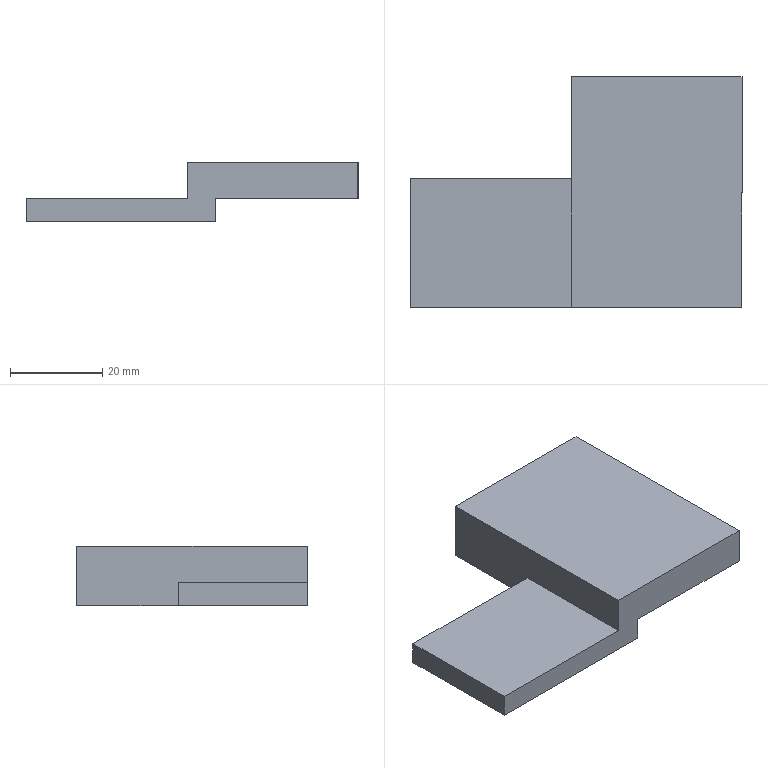Component | SolidWorks | MirroredGripper-2024-3-4-06-2 | 1 solid | 11 faces | box 72 x 50 x 13 mm | volume 21200 mm3 | plane 11 | material S45C
STEP:
#1=COLOUR_RGB('',0.7922,0.8196,0.9333);
#2=FILL_AREA_STYLE_COLOUR('',#1);
#3=FILL_AREA_STYLE('',(#2));
#4=SURFACE_STYLE_FILL_AREA(#3);
#5=SURFACE_SIDE_STYLE('',(#4));
#6=SURFACE_STYLE_USAGE(.BOTH.,#5);
#7=PRESENTATION_STYLE_ASSIGNMENT((#6));
#8=CARTESIAN_POINT('',(-6.049,-0.2645,10.276));
#9=VERTEX_POINT('',#8);
#10=CARTESIAN_POINT('',(-6.049,0.8378,10.276));
#11=VERTEX_POINT('',#10);
#12=CARTESIAN_POINT('',(-6.049,-0.2645,10.276));
#13=DIRECTION('',(0.,1.,-0.));
#14=VECTOR('',#13,39.37);
#15=LINE('',#12,#14);
#16=EDGE_CURVE('',#9,#11,#15,.T.);
#17=ORIENTED_EDGE('',*,*,#16,.F.);
#18=CARTESIAN_POINT('',(-6.049,-0.2645,10.472));
#19=VERTEX_POINT('',#18);
#20=CARTESIAN_POINT('',(-6.049,-0.2645,10.472));
#21=DIRECTION('',(-0.,0.,1.));
#22=VECTOR('',#21,39.37);
#23=LINE('',#20,#22);
#24=EDGE_CURVE('',#9,#19,#23,.T.);
#25=ORIENTED_EDGE('',*,*,#24,.T.);
#26=CARTESIAN_POINT('',(-6.049,0.8378,10.472));
#27=VERTEX_POINT('',#26);
#28=CARTESIAN_POINT('',(-6.049,-0.2645,10.472));
#29=DIRECTION('',(0.,1.,-0.));
#30=VECTOR('',#29,39.37);
#31=LINE('',#28,#30);
#32=EDGE_CURVE('',#19,#27,#31,.T.);
#33=ORIENTED_EDGE('',*,*,#32,.T.);
#34=CARTESIAN_POINT('',(-6.049,0.8378,11.85));
#35=DIRECTION('',(0.,-0.,-1.));
#36=VECTOR('',#35,39.37);
#37=LINE('',#34,#36);
#38=EDGE_CURVE('',#27,#11,#37,.T.);
#39=ORIENTED_EDGE('',*,*,#38,.T.);
#40=EDGE_LOOP('',(#17,#25,#33,#39));
#41=FACE_OUTER_BOUND('',#40,.T.);
#42=CARTESIAN_POINT('',(-6.049,-0.2645,10.472));
#43=DIRECTION('',(1.,-0.,0.));
#44=DIRECTION('',(0.,1.,-0.));
#45=AXIS2_PLACEMENT_3D('',#42,#43,#44);
#46=PLANE('',#45);
#47=ADVANCED_FACE('',(#41),#46,.F.);
#48=ORIENTED_EDGE('',*,*,#32,.F.);
#49=CARTESIAN_POINT('',(-4.671,-0.2645,10.472));
#50=VERTEX_POINT('',#49);
#51=CARTESIAN_POINT('',(-6.049,-0.2645,10.472));
#52=DIRECTION('',(1.,-0.,0.));
#53=VECTOR('',#52,39.37);
#54=LINE('',#51,#53);
#55=EDGE_CURVE('',#19,#50,#54,.T.);
#56=ORIENTED_EDGE('',*,*,#55,.T.);
#57=CARTESIAN_POINT('',(-4.671,0.8378,10.472));
#58=VERTEX_POINT('',#57);
#59=CARTESIAN_POINT('',(-4.671,-0.2645,10.472));
#60=DIRECTION('',(0.,1.,-0.));
#61=VECTOR('',#60,39.37);
#62=LINE('',#59,#61);
#63=EDGE_CURVE('',#50,#58,#62,.T.);
#64=ORIENTED_EDGE('',*,*,#63,.T.);
#65=CARTESIAN_POINT('',(-6.049,0.8378,10.472));
#66=DIRECTION('',(1.,-0.,0.));
#67=VECTOR('',#66,39.37);
#68=LINE('',#65,#67);
#69=EDGE_CURVE('',#27,#58,#68,.T.);
#70=ORIENTED_EDGE('',*,*,#69,.F.);
#71=EDGE_LOOP('',(#48,#56,#64,#70));
#72=FACE_OUTER_BOUND('',#71,.T.);
#73=CARTESIAN_POINT('',(-6.049,-0.2645,10.472));
#74=DIRECTION('',(0.,-0.,-1.));
#75=DIRECTION('',(-0.,-1.,0.));
#76=AXIS2_PLACEMENT_3D('',#73,#74,#75);
#77=PLANE('',#76);
#78=ADVANCED_FACE('',(#72),#77,.F.);
#79=ORIENTED_EDGE('',*,*,#63,.F.);
#80=CARTESIAN_POINT('',(-4.671,-0.2645,10.787));
#81=VERTEX_POINT('',#80);
#82=CARTESIAN_POINT('',(-4.671,-0.2645,10.472));
#83=DIRECTION('',(-0.,0.,1.));
#84=VECTOR('',#83,39.37);
#85=LINE('',#82,#84);
#86=EDGE_CURVE('',#50,#81,#85,.T.);
#87=ORIENTED_EDGE('',*,*,#86,.T.);
#88=CARTESIAN_POINT('',(-4.671,1.704,10.787));
#89=VERTEX_POINT('',#88);
#90=CARTESIAN_POINT('',(-4.671,-0.2645,10.787));
#91=DIRECTION('',(0.,1.,-0.));
#92=VECTOR('',#91,39.37);
#93=LINE('',#90,#92);
#94=EDGE_CURVE('',#81,#89,#93,.T.);
#95=ORIENTED_EDGE('',*,*,#94,.T.);
#96=CARTESIAN_POINT('',(-4.671,1.704,10.276));
#97=VERTEX_POINT('',#96);
#98=CARTESIAN_POINT('',(-4.671,1.704,10.472));
#99=DIRECTION('',(-0.,0.,1.));
#100=VECTOR('',#99,39.37);
#101=LINE('',#98,#100);
#102=EDGE_CURVE('',#97,#89,#101,.T.);
#103=ORIENTED_EDGE('',*,*,#102,.F.);
#104=CARTESIAN_POINT('',(-4.671,0.8378,10.276));
#105=VERTEX_POINT('',#104);
#106=CARTESIAN_POINT('',(-4.671,1.704,10.276));
#107=DIRECTION('',(0.,1.,-0.));
#108=VECTOR('',#107,39.37);
#109=LINE('',#106,#108);
#110=EDGE_CURVE('',#105,#97,#109,.T.);
#111=ORIENTED_EDGE('',*,*,#110,.F.);
#112=CARTESIAN_POINT('',(-4.671,0.8378,11.85));
#113=DIRECTION('',(0.,-0.,-1.));
#114=VECTOR('',#113,39.37);
#115=LINE('',#112,#114);
#116=EDGE_CURVE('',#58,#105,#115,.T.);
#117=ORIENTED_EDGE('',*,*,#116,.F.);
#118=EDGE_LOOP('',(#79,#87,#95,#103,#111,#117));
#119=FACE_OUTER_BOUND('',#118,.T.);
#120=CARTESIAN_POINT('',(-4.671,-0.2645,10.472));
#121=DIRECTION('',(1.,-0.,0.));
#122=DIRECTION('',(0.,1.,-0.));
#123=AXIS2_PLACEMENT_3D('',#120,#121,#122);
#124=PLANE('',#123);
#125=ADVANCED_FACE('',(#119),#124,.F.);
#126=CARTESIAN_POINT('',(-3.215,1.704,10.787));
#127=VERTEX_POINT('',#126);
#128=CARTESIAN_POINT('',(-4.671,1.704,10.787));
#129=DIRECTION('',(1.,-0.,0.));
#130=VECTOR('',#129,39.37);
#131=LINE('',#128,#130);
#132=EDGE_CURVE('',#89,#127,#131,.T.);
#133=ORIENTED_EDGE('',*,*,#132,.F.);
#134=ORIENTED_EDGE('',*,*,#94,.F.);
#135=CARTESIAN_POINT('',(-3.215,-0.2645,10.787));
#136=VERTEX_POINT('',#135);
#137=CARTESIAN_POINT('',(-4.671,-0.2645,10.787));
#138=DIRECTION('',(1.,-0.,0.));
#139=VECTOR('',#138,39.37);
#140=LINE('',#137,#139);
#141=EDGE_CURVE('',#81,#136,#140,.T.);
#142=ORIENTED_EDGE('',*,*,#141,.T.);
#143=CARTESIAN_POINT('',(-3.215,-0.2645,10.787));
#144=DIRECTION('',(0.,1.,-0.));
#145=VECTOR('',#144,39.37);
#146=LINE('',#143,#145);
#147=EDGE_CURVE('',#136,#127,#146,.T.);
#148=ORIENTED_EDGE('',*,*,#147,.T.);
#149=EDGE_LOOP('',(#133,#134,#142,#148));
#150=FACE_OUTER_BOUND('',#149,.T.);
#151=CARTESIAN_POINT('',(-4.671,-0.2645,10.787));
#152=DIRECTION('',(0.,-0.,-1.));
#153=DIRECTION('',(-0.,-1.,0.));
#154=AXIS2_PLACEMENT_3D('',#151,#152,#153);
#155=PLANE('',#154);
#156=ADVANCED_FACE('',(#150),#155,.F.);
#157=CARTESIAN_POINT('',(-3.215,1.704,10.472));
#158=VERTEX_POINT('',#157);
#159=CARTESIAN_POINT('',(-3.215,1.704,10.472));
#160=DIRECTION('',(0.,-0.,-1.));
#161=VECTOR('',#160,39.37);
#162=LINE('',#159,#161);
#163=EDGE_CURVE('',#127,#158,#162,.T.);
#164=ORIENTED_EDGE('',*,*,#163,.F.);
#165=ORIENTED_EDGE('',*,*,#147,.F.);
#166=CARTESIAN_POINT('',(-3.215,-0.2645,10.472));
#167=VERTEX_POINT('',#166);
#168=CARTESIAN_POINT('',(-3.215,-0.2645,10.472));
#169=DIRECTION('',(0.,-0.,-1.));
#170=VECTOR('',#169,39.37);
#171=LINE('',#168,#170);
#172=EDGE_CURVE('',#136,#167,#171,.T.);
#173=ORIENTED_EDGE('',*,*,#172,.T.);
#174=CARTESIAN_POINT('',(-3.215,-0.2645,10.472));
#175=DIRECTION('',(0.,1.,-0.));
#176=VECTOR('',#175,39.37);
#177=LINE('',#174,#176);
#178=EDGE_CURVE('',#167,#158,#177,.T.);
#179=ORIENTED_EDGE('',*,*,#178,.T.);
#180=EDGE_LOOP('',(#164,#165,#173,#179));
#181=FACE_OUTER_BOUND('',#180,.T.);
#182=CARTESIAN_POINT('',(-3.215,-0.2645,10.472));
#183=DIRECTION('',(-1.,0.,-0.));
#184=DIRECTION('',(-0.,-1.,0.));
#185=AXIS2_PLACEMENT_3D('',#182,#183,#184);
#186=PLANE('',#185);
#187=ADVANCED_FACE('',(#181),#186,.F.);
#188=CARTESIAN_POINT('',(-4.435,1.704,10.472));
#189=VERTEX_POINT('',#188);
#190=CARTESIAN_POINT('',(-4.435,1.704,10.472));
#191=DIRECTION('',(-1.,0.,-0.));
#192=VECTOR('',#191,39.37);
#193=LINE('',#190,#192);
#194=EDGE_CURVE('',#158,#189,#193,.T.);
#195=ORIENTED_EDGE('',*,*,#194,.F.);
#196=ORIENTED_EDGE('',*,*,#178,.F.);
#197=CARTESIAN_POINT('',(-4.435,-0.2645,10.472));
#198=VERTEX_POINT('',#197);
#199=CARTESIAN_POINT('',(-4.435,-0.2645,10.472));
#200=DIRECTION('',(-1.,0.,-0.));
#201=VECTOR('',#200,39.37);
#202=LINE('',#199,#201);
#203=EDGE_CURVE('',#167,#198,#202,.T.);
#204=ORIENTED_EDGE('',*,*,#203,.T.);
#205=CARTESIAN_POINT('',(-4.435,-0.2645,10.472));
#206=DIRECTION('',(0.,1.,-0.));
#207=VECTOR('',#206,39.37);
#208=LINE('',#205,#207);
#209=EDGE_CURVE('',#198,#189,#208,.T.);
#210=ORIENTED_EDGE('',*,*,#209,.T.);
#211=EDGE_LOOP('',(#195,#196,#204,#210));
#212=FACE_OUTER_BOUND('',#211,.T.);
#213=CARTESIAN_POINT('',(-4.435,-0.2645,10.472));
#214=DIRECTION('',(-0.,0.,1.));
#215=DIRECTION('',(0.,1.,-0.));
#216=AXIS2_PLACEMENT_3D('',#213,#214,#215);
#217=PLANE('',#216);
#218=ADVANCED_FACE('',(#212),#217,.F.);
#219=CARTESIAN_POINT('',(-4.435,1.704,10.276));
#220=VERTEX_POINT('',#219);
#221=CARTESIAN_POINT('',(-4.435,1.704,10.472));
#222=DIRECTION('',(0.,-0.,-1.));
#223=VECTOR('',#222,39.37);
#224=LINE('',#221,#223);
#225=EDGE_CURVE('',#189,#220,#224,.T.);
#226=ORIENTED_EDGE('',*,*,#225,.F.);
#227=ORIENTED_EDGE('',*,*,#209,.F.);
#228=CARTESIAN_POINT('',(-4.435,-0.2645,10.276));
#229=VERTEX_POINT('',#228);
#230=CARTESIAN_POINT('',(-4.435,-0.2645,10.472));
#231=DIRECTION('',(0.,-0.,-1.));
#232=VECTOR('',#231,39.37);
#233=LINE('',#230,#232);
#234=EDGE_CURVE('',#198,#229,#233,.T.);
#235=ORIENTED_EDGE('',*,*,#234,.T.);
#236=CARTESIAN_POINT('',(-4.435,-0.2645,10.276));
#237=DIRECTION('',(0.,1.,-0.));
#238=VECTOR('',#237,39.37);
#239=LINE('',#236,#238);
#240=EDGE_CURVE('',#229,#220,#239,.T.);
#241=ORIENTED_EDGE('',*,*,#240,.T.);
#242=EDGE_LOOP('',(#226,#227,#235,#241));
#243=FACE_OUTER_BOUND('',#242,.T.);
#244=CARTESIAN_POINT('',(-4.435,-0.2645,10.472));
#245=DIRECTION('',(-1.,0.,-0.));
#246=DIRECTION('',(-0.,-1.,0.));
#247=AXIS2_PLACEMENT_3D('',#244,#245,#246);
#248=PLANE('',#247);
#249=ADVANCED_FACE('',(#243),#248,.F.);
#250=CARTESIAN_POINT('',(-6.049,1.704,10.276));
#251=DIRECTION('',(-1.,0.,-0.));
#252=VECTOR('',#251,39.37);
#253=LINE('',#250,#252);
#254=EDGE_CURVE('',#220,#97,#253,.T.);
#255=ORIENTED_EDGE('',*,*,#254,.F.);
#256=ORIENTED_EDGE('',*,*,#240,.F.);
#257=CARTESIAN_POINT('',(-6.049,-0.2645,10.276));
#258=DIRECTION('',(-1.,0.,-0.));
#259=VECTOR('',#258,39.37);
#260=LINE('',#257,#259);
#261=EDGE_CURVE('',#229,#9,#260,.T.);
#262=ORIENTED_EDGE('',*,*,#261,.T.);
#263=ORIENTED_EDGE('',*,*,#16,.T.);
#264=CARTESIAN_POINT('',(-6.049,0.8378,10.276));
#265=DIRECTION('',(1.,-0.,0.));
#266=VECTOR('',#265,39.37);
#267=LINE('',#264,#266);
#268=EDGE_CURVE('',#11,#105,#267,.T.);
#269=ORIENTED_EDGE('',*,*,#268,.T.);
#270=ORIENTED_EDGE('',*,*,#110,.T.);
#271=EDGE_LOOP('',(#255,#256,#262,#263,#269,#270));
#272=FACE_OUTER_BOUND('',#271,.T.);
#273=CARTESIAN_POINT('',(-6.049,-0.2645,10.276));
#274=DIRECTION('',(-0.,0.,1.));
#275=DIRECTION('',(0.,1.,-0.));
#276=AXIS2_PLACEMENT_3D('',#273,#274,#275);
#277=PLANE('',#276);
#278=ADVANCED_FACE('',(#272),#277,.F.);
#279=ORIENTED_EDGE('',*,*,#24,.F.);
#280=ORIENTED_EDGE('',*,*,#261,.F.);
#281=ORIENTED_EDGE('',*,*,#234,.F.);
#282=ORIENTED_EDGE('',*,*,#203,.F.);
#283=ORIENTED_EDGE('',*,*,#172,.F.);
#284=ORIENTED_EDGE('',*,*,#141,.F.);
#285=ORIENTED_EDGE('',*,*,#86,.F.);
#286=ORIENTED_EDGE('',*,*,#55,.F.);
#287=EDGE_LOOP('',(#279,#280,#281,#282,#283,#284,#285,#286));
#288=FACE_OUTER_BOUND('',#287,.T.);
#289=CARTESIAN_POINT('',(-6.049,-0.2645,10.472));
#290=DIRECTION('',(0.,1.,-0.));
#291=DIRECTION('',(-1.,0.,-0.));
#292=AXIS2_PLACEMENT_3D('',#289,#290,#291);
#293=PLANE('',#292);
#294=ADVANCED_FACE('',(#288),#293,.F.);
#295=ORIENTED_EDGE('',*,*,#102,.T.);
#296=ORIENTED_EDGE('',*,*,#132,.T.);
#297=ORIENTED_EDGE('',*,*,#163,.T.);
#298=ORIENTED_EDGE('',*,*,#194,.T.);
#299=ORIENTED_EDGE('',*,*,#225,.T.);
#300=ORIENTED_EDGE('',*,*,#254,.T.);
#301=EDGE_LOOP('',(#295,#296,#297,#298,#299,#300));
#302=FACE_OUTER_BOUND('',#301,.T.);
#303=CARTESIAN_POINT('',(-6.049,1.704,10.472));
#304=DIRECTION('',(0.,1.,-0.));
#305=DIRECTION('',(-1.,0.,-0.));
#306=AXIS2_PLACEMENT_3D('',#303,#304,#305);
#307=PLANE('',#306);
#308=ADVANCED_FACE('',(#302),#307,.T.);
#309=ORIENTED_EDGE('',*,*,#38,.F.);
#310=ORIENTED_EDGE('',*,*,#69,.T.);
#311=ORIENTED_EDGE('',*,*,#116,.T.);
#312=ORIENTED_EDGE('',*,*,#268,.F.);
#313=EDGE_LOOP('',(#309,#310,#311,#312));
#314=FACE_OUTER_BOUND('',#313,.T.);
#315=CARTESIAN_POINT('',(-6.049,0.8378,11.85));
#316=DIRECTION('',(-0.,-1.,0.));
#317=DIRECTION('',(1.,-0.,0.));
#318=AXIS2_PLACEMENT_3D('',#315,#316,#317);
#319=PLANE('',#318);
#320=ADVANCED_FACE('',(#314),#319,.F.);
#321=CLOSED_SHELL('',(#47,#78,#125,#156,#187,#218,#249,#278,#294,#308,#320));
#322=MANIFOLD_SOLID_BREP('',#321);
#323=STYLED_ITEM('',(#7),#322);
#324=PRESENTATION_LAYER_ASSIGNMENT('','',(#323));
#325=CARTESIAN_POINT('',(0.,0.,0.));
#326=DIRECTION('',(0.,0.,1.));
#327=DIRECTION('',(1.,0.,0.));
#328=AXIS2_PLACEMENT_3D('',#325,#326,#327);
#329=(LENGTH_UNIT()NAMED_UNIT(*)SI_UNIT($,.METRE.));
#330=LENGTH_MEASURE_WITH_UNIT(LENGTH_MEASURE(0.0254),#329);
#331=DIMENSIONAL_EXPONENTS(1.,0.,0.,0.,0.,0.,0.);
#332=(CONVERSION_BASED_UNIT('',#330)LENGTH_UNIT()NAMED_UNIT(#331));
#333=UNCERTAINTY_MEASURE_WITH_UNIT(LENGTH_MEASURE(0.00001),#332,'','');
#334=(NAMED_UNIT(*)PLANE_ANGLE_UNIT()SI_UNIT($,.RADIAN.));
#335=(NAMED_UNIT(*)SI_UNIT($,.STERADIAN.)SOLID_ANGLE_UNIT());
#336=(GEOMETRIC_REPRESENTATION_CONTEXT(3)GLOBAL_UNCERTAINTY_ASSIGNED_CONTEXT((#333))GLOBAL_UNIT_ASSIGNED_CONTEXT((#332,#334,#335))REPRESENTATION_CONTEXT('',''));
#337=ADVANCED_BREP_SHAPE_REPRESENTATION('',(#322,#328),#336);
#338=(LENGTH_UNIT()NAMED_UNIT(*)SI_UNIT($,.METRE.));
#339=LENGTH_MEASURE_WITH_UNIT(LENGTH_MEASURE(0.0254),#338);
#340=DIMENSIONAL_EXPONENTS(1.,0.,0.,0.,0.,0.,0.);
#341=(CONVERSION_BASED_UNIT('',#339)LENGTH_UNIT()NAMED_UNIT(#340));
#342=UNCERTAINTY_MEASURE_WITH_UNIT(LENGTH_MEASURE(0.00001),#341,'','');
#343=(NAMED_UNIT(*)PLANE_ANGLE_UNIT()SI_UNIT($,.RADIAN.));
#344=(NAMED_UNIT(*)SI_UNIT($,.STERADIAN.)SOLID_ANGLE_UNIT());
#345=(GEOMETRIC_REPRESENTATION_CONTEXT(3)GLOBAL_UNCERTAINTY_ASSIGNED_CONTEXT((#342))GLOBAL_UNIT_ASSIGNED_CONTEXT((#341,#343,#344))REPRESENTATION_CONTEXT('',''));
#346=MECHANICAL_DESIGN_GEOMETRIC_PRESENTATION_REPRESENTATION('',(#323),#345);